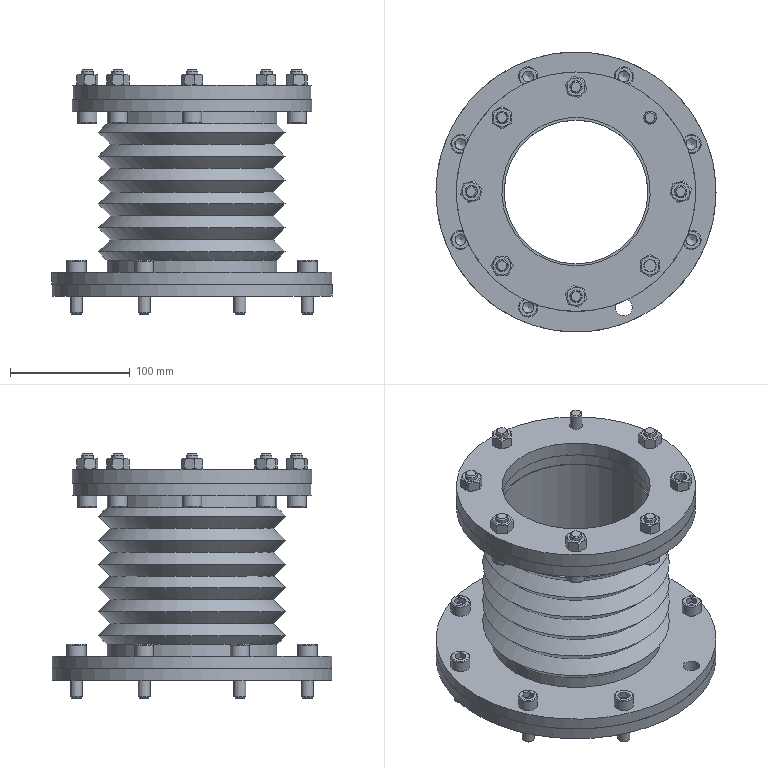Assembly | NX | mm | 26 component files | 26 solids | 448 faces | box 234 x 234 x 204 mm | volume 1634384 mm3 | plane 282 | cylinder 84 | cone 68 | torus 14 | commonest cylinder face diameters 10 x21 11 x16 14 x16 16 x14 200 x2 234 x2 126 x2 150 x2
Bill of materials:
GB_T70_1_M10X35 | 14 |  | Socket-head cap screw form: cylindrical head with a hexagonal socket on top, a plain cylindrical shank of smaller diameter, and a small chamfer at the shank end.
CH3404-1 | 1 |  | Flat circular annular plate with a large central bore and 8 small through-holes on a bolt circle. In plan view, the holes are offset so none sits on the vertical or horizontal axis.
CH3404.8.2-2 | 1 |  | Flat circular annular plate with a large central bore and 8 small through-holes on a bolt circle. In plan view, holes sit on the vertical and horizontal axes. It is thicker relative to diameter than parts 1 and 5.
GB_T41-2000 | 7 |  | Hexagonal nut form: hex prism with a plain cylindrical through-bore and chamfered corners on both end faces.
CH3404.9-2 | 1 |  | Thin-walled hollow cylindrical sleeve. The outside has 6 V-profile ridges along most of its length, with plain cylindrical bands at both ends.
CH3404.9-3 | 1 |  | Flat circular annular plate with a large central bore and 8 small through-holes on a bolt circle. In plan view, the holes are offset from the vertical and horizontal axes.
CH3404.9-1 | 1 |  | Flat circular annular plate with a large central bore, 8 small through-holes on a bolt circle (on the axes in plan view), and a shallow concentric step or recess ring around the bore on one face.
Mates:
1. touch align | CH3404_9-1 1 datumplane | assembly datumplane
2. touch align | CH3404_9-1 1 datumplane | assembly datumplane
3. touch align | CH3404_9-1 1 face | assembly datumaxis
4. touch align | CH3404_9-2 1 face | CH3404_9-1 1 face
5. touch align | CH3404_9-2 1 | assembly datumplane
6. touch align | CH3404_9-2 1 face | assembly datumaxis
7. touch align | CH3404_9-3 1 datumplane | assembly datumplane
8. touch align | CH3404_9-3 1 face | CH3404_9-2 1 face
9. touch align | CH3404_9-3 1 face | assembly datumaxis
10. touch align | CH3404-1 1 face | CH3404_9-3 1 face